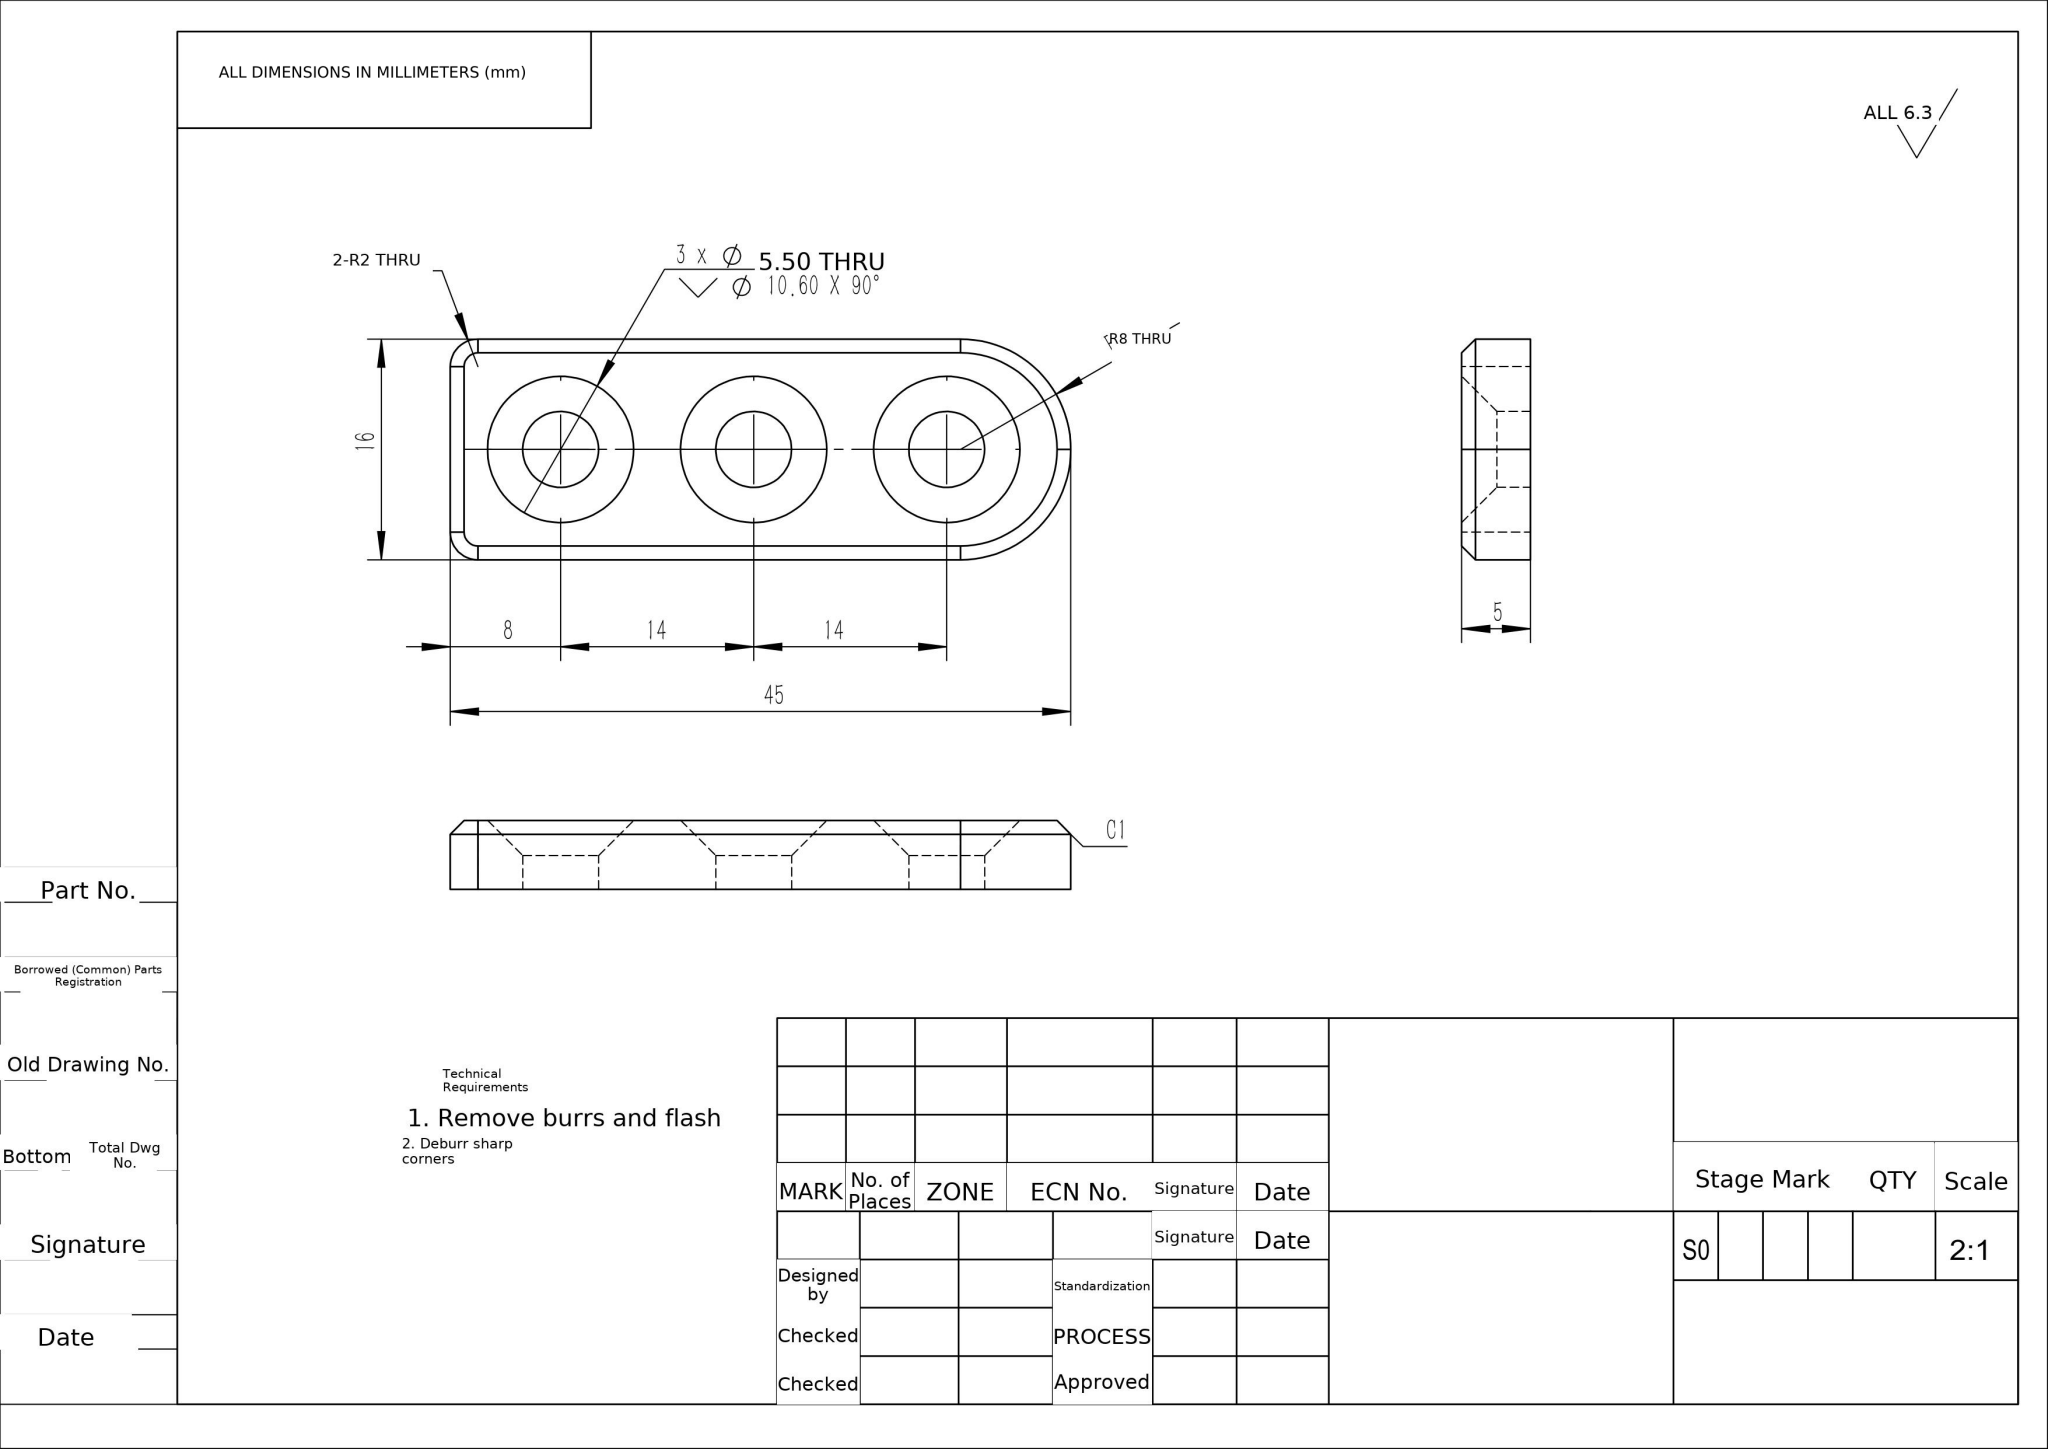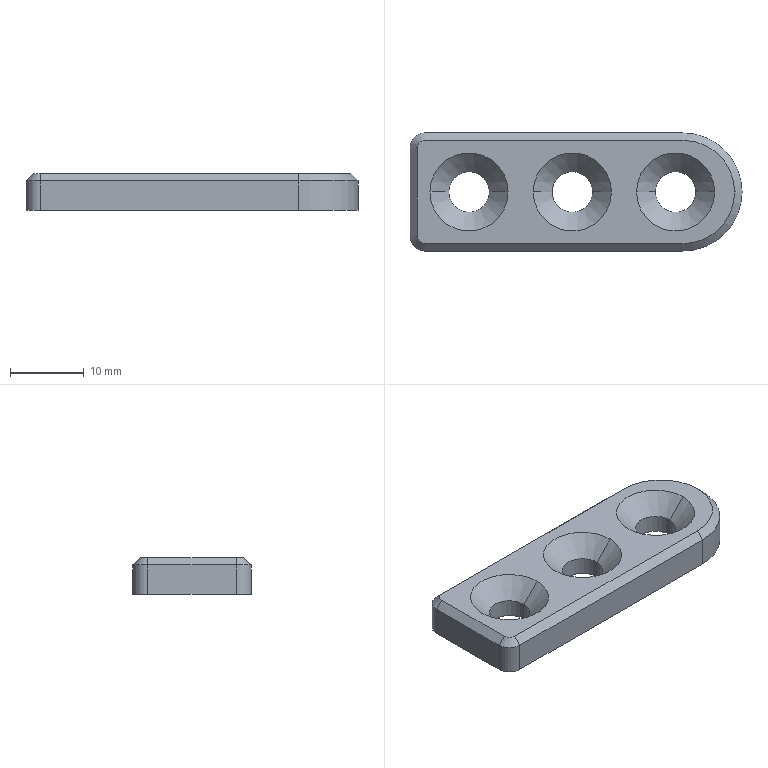Part | NX | mm | 1 solid | 28 faces | box 45 x 16 x 5 mm | volume 2821 mm3 | cone 10 | cylinder 10 | plane 8 | commonest cylinder face diameters 5.5 x6 16 x2 4 x2
STEP:
#1=COLOUR_RGB('',0.502,1.,1.);
#2=FILL_AREA_STYLE_COLOUR('',#1);
#3=FILL_AREA_STYLE('',(#2));
#4=SURFACE_STYLE_FILL_AREA(#3);
#5=SURFACE_SIDE_STYLE('',(#4));
#6=SURFACE_STYLE_USAGE(.BOTH.,#5);
#7=PRESENTATION_STYLE_ASSIGNMENT((#6));
#8=CARTESIAN_POINT('',(5.25,8.,2.45));
#9=VERTEX_POINT('',#8);
#10=CARTESIAN_POINT('',(10.75,8.,2.45));
#11=VERTEX_POINT('',#10);
#12=CARTESIAN_POINT('',(8.,8.,2.45));
#13=DIRECTION('',(0.,0.,1.));
#14=DIRECTION('',(1.,0.,0.));
#15=AXIS2_PLACEMENT_3D('',#12,#13,#14);
#16=CIRCLE('',#15,2.75);
#17=EDGE_CURVE('',#9,#11,#16,.T.);
#18=ORIENTED_EDGE('',*,*,#17,.F.);
#19=CARTESIAN_POINT('',(2.7,8.,5.));
#20=VERTEX_POINT('',#19);
#21=CARTESIAN_POINT('',(2.7,8.,5.));
#22=DIRECTION('',(-0.7071,0.,0.7071));
#23=VECTOR('',#22,1000.);
#24=LINE('',#21,#23);
#25=EDGE_CURVE('',#9,#20,#24,.T.);
#26=ORIENTED_EDGE('',*,*,#25,.T.);
#27=CARTESIAN_POINT('',(13.3,8.,5.));
#28=VERTEX_POINT('',#27);
#29=CARTESIAN_POINT('',(8.,8.,5.));
#30=DIRECTION('',(0.,0.,1.));
#31=DIRECTION('',(1.,0.,0.));
#32=AXIS2_PLACEMENT_3D('',#29,#30,#31);
#33=CIRCLE('',#32,5.3);
#34=EDGE_CURVE('',#20,#28,#33,.T.);
#35=ORIENTED_EDGE('',*,*,#34,.T.);
#36=CARTESIAN_POINT('',(13.3,8.,5.));
#37=DIRECTION('',(0.7071,0.,0.7071));
#38=VECTOR('',#37,1000.);
#39=LINE('',#36,#38);
#40=EDGE_CURVE('',#11,#28,#39,.T.);
#41=ORIENTED_EDGE('',*,*,#40,.F.);
#42=EDGE_LOOP('',(#18,#26,#35,#41));
#43=FACE_OUTER_BOUND('',#42,.T.);
#44=CARTESIAN_POINT('',(8.,8.,5.));
#45=DIRECTION('',(0.,0.,1.));
#46=DIRECTION('',(1.,0.,0.));
#47=AXIS2_PLACEMENT_3D('',#44,#45,#46);
#48=CONICAL_SURFACE('',#47,5.3,0.7854);
#49=ADVANCED_FACE('',(#43),#48,.F.);
#50=CARTESIAN_POINT('',(19.25,8.,2.45));
#51=VERTEX_POINT('',#50);
#52=CARTESIAN_POINT('',(24.75,8.,2.45));
#53=VERTEX_POINT('',#52);
#54=CARTESIAN_POINT('',(22.,8.,2.45));
#55=DIRECTION('',(0.,0.,1.));
#56=DIRECTION('',(1.,0.,0.));
#57=AXIS2_PLACEMENT_3D('',#54,#55,#56);
#58=CIRCLE('',#57,2.75);
#59=EDGE_CURVE('',#51,#53,#58,.T.);
#60=ORIENTED_EDGE('',*,*,#59,.F.);
#61=CARTESIAN_POINT('',(16.7,8.,5.));
#62=VERTEX_POINT('',#61);
#63=CARTESIAN_POINT('',(16.7,8.,5.));
#64=DIRECTION('',(-0.7071,0.,0.7071));
#65=VECTOR('',#64,1000.);
#66=LINE('',#63,#65);
#67=EDGE_CURVE('',#51,#62,#66,.T.);
#68=ORIENTED_EDGE('',*,*,#67,.T.);
#69=CARTESIAN_POINT('',(27.3,8.,5.));
#70=VERTEX_POINT('',#69);
#71=CARTESIAN_POINT('',(22.,8.,5.));
#72=DIRECTION('',(0.,0.,1.));
#73=DIRECTION('',(1.,0.,0.));
#74=AXIS2_PLACEMENT_3D('',#71,#72,#73);
#75=CIRCLE('',#74,5.3);
#76=EDGE_CURVE('',#62,#70,#75,.T.);
#77=ORIENTED_EDGE('',*,*,#76,.T.);
#78=CARTESIAN_POINT('',(27.3,8.,5.));
#79=DIRECTION('',(0.7071,0.,0.7071));
#80=VECTOR('',#79,1000.);
#81=LINE('',#78,#80);
#82=EDGE_CURVE('',#53,#70,#81,.T.);
#83=ORIENTED_EDGE('',*,*,#82,.F.);
#84=EDGE_LOOP('',(#60,#68,#77,#83));
#85=FACE_OUTER_BOUND('',#84,.T.);
#86=CARTESIAN_POINT('',(22.,8.,5.));
#87=DIRECTION('',(0.,0.,1.));
#88=DIRECTION('',(1.,0.,0.));
#89=AXIS2_PLACEMENT_3D('',#86,#87,#88);
#90=CONICAL_SURFACE('',#89,5.3,0.7854);
#91=ADVANCED_FACE('',(#85),#90,.F.);
#92=CARTESIAN_POINT('',(33.25,8.,2.45));
#93=VERTEX_POINT('',#92);
#94=CARTESIAN_POINT('',(38.75,8.,2.45));
#95=VERTEX_POINT('',#94);
#96=CARTESIAN_POINT('',(36.,8.,2.45));
#97=DIRECTION('',(0.,0.,1.));
#98=DIRECTION('',(1.,0.,0.));
#99=AXIS2_PLACEMENT_3D('',#96,#97,#98);
#100=CIRCLE('',#99,2.75);
#101=EDGE_CURVE('',#93,#95,#100,.T.);
#102=ORIENTED_EDGE('',*,*,#101,.F.);
#103=CARTESIAN_POINT('',(30.7,8.,5.));
#104=VERTEX_POINT('',#103);
#105=CARTESIAN_POINT('',(30.7,8.,5.));
#106=DIRECTION('',(-0.7071,0.,0.7071));
#107=VECTOR('',#106,1000.);
#108=LINE('',#105,#107);
#109=EDGE_CURVE('',#93,#104,#108,.T.);
#110=ORIENTED_EDGE('',*,*,#109,.T.);
#111=CARTESIAN_POINT('',(41.3,8.,5.));
#112=VERTEX_POINT('',#111);
#113=CARTESIAN_POINT('',(36.,8.,5.));
#114=DIRECTION('',(0.,0.,1.));
#115=DIRECTION('',(1.,0.,0.));
#116=AXIS2_PLACEMENT_3D('',#113,#114,#115);
#117=CIRCLE('',#116,5.3);
#118=EDGE_CURVE('',#104,#112,#117,.T.);
#119=ORIENTED_EDGE('',*,*,#118,.T.);
#120=CARTESIAN_POINT('',(41.3,8.,5.));
#121=DIRECTION('',(0.7071,0.,0.7071));
#122=VECTOR('',#121,1000.);
#123=LINE('',#120,#122);
#124=EDGE_CURVE('',#95,#112,#123,.T.);
#125=ORIENTED_EDGE('',*,*,#124,.F.);
#126=EDGE_LOOP('',(#102,#110,#119,#125));
#127=FACE_OUTER_BOUND('',#126,.T.);
#128=CARTESIAN_POINT('',(36.,8.,5.));
#129=DIRECTION('',(0.,0.,1.));
#130=DIRECTION('',(1.,0.,0.));
#131=AXIS2_PLACEMENT_3D('',#128,#129,#130);
#132=CONICAL_SURFACE('',#131,5.3,0.7854);
#133=ADVANCED_FACE('',(#127),#132,.F.);
#134=CARTESIAN_POINT('',(33.25,8.,0.));
#135=VERTEX_POINT('',#134);
#136=CARTESIAN_POINT('',(38.75,8.,0.));
#137=VERTEX_POINT('',#136);
#138=CARTESIAN_POINT('',(36.,8.,0.));
#139=DIRECTION('',(0.,0.,1.));
#140=DIRECTION('',(1.,0.,0.));
#141=AXIS2_PLACEMENT_3D('',#138,#139,#140);
#142=CIRCLE('',#141,2.75);
#143=EDGE_CURVE('',#135,#137,#142,.T.);
#144=ORIENTED_EDGE('',*,*,#143,.F.);
#145=CARTESIAN_POINT('',(33.25,8.,0.));
#146=DIRECTION('',(0.,0.,1.));
#147=VECTOR('',#146,1000.);
#148=LINE('',#145,#147);
#149=EDGE_CURVE('',#135,#93,#148,.T.);
#150=ORIENTED_EDGE('',*,*,#149,.T.);
#151=ORIENTED_EDGE('',*,*,#101,.T.);
#152=CARTESIAN_POINT('',(38.75,8.,0.));
#153=DIRECTION('',(0.,0.,1.));
#154=VECTOR('',#153,1000.);
#155=LINE('',#152,#154);
#156=EDGE_CURVE('',#137,#95,#155,.T.);
#157=ORIENTED_EDGE('',*,*,#156,.F.);
#158=EDGE_LOOP('',(#144,#150,#151,#157));
#159=FACE_OUTER_BOUND('',#158,.T.);
#160=CARTESIAN_POINT('',(36.,8.,0.));
#161=DIRECTION('',(0.,0.,1.));
#162=DIRECTION('',(1.,0.,0.));
#163=AXIS2_PLACEMENT_3D('',#160,#161,#162);
#164=CYLINDRICAL_SURFACE('',#163,2.75);
#165=ADVANCED_FACE('',(#159),#164,.F.);
#166=CARTESIAN_POINT('',(19.25,8.,0.));
#167=VERTEX_POINT('',#166);
#168=CARTESIAN_POINT('',(24.75,8.,0.));
#169=VERTEX_POINT('',#168);
#170=CARTESIAN_POINT('',(22.,8.,0.));
#171=DIRECTION('',(0.,0.,1.));
#172=DIRECTION('',(1.,0.,0.));
#173=AXIS2_PLACEMENT_3D('',#170,#171,#172);
#174=CIRCLE('',#173,2.75);
#175=EDGE_CURVE('',#167,#169,#174,.T.);
#176=ORIENTED_EDGE('',*,*,#175,.F.);
#177=CARTESIAN_POINT('',(19.25,8.,0.));
#178=DIRECTION('',(0.,0.,1.));
#179=VECTOR('',#178,1000.);
#180=LINE('',#177,#179);
#181=EDGE_CURVE('',#167,#51,#180,.T.);
#182=ORIENTED_EDGE('',*,*,#181,.T.);
#183=ORIENTED_EDGE('',*,*,#59,.T.);
#184=CARTESIAN_POINT('',(24.75,8.,0.));
#185=DIRECTION('',(0.,0.,1.));
#186=VECTOR('',#185,1000.);
#187=LINE('',#184,#186);
#188=EDGE_CURVE('',#169,#53,#187,.T.);
#189=ORIENTED_EDGE('',*,*,#188,.F.);
#190=EDGE_LOOP('',(#176,#182,#183,#189));
#191=FACE_OUTER_BOUND('',#190,.T.);
#192=CARTESIAN_POINT('',(22.,8.,0.));
#193=DIRECTION('',(0.,0.,1.));
#194=DIRECTION('',(1.,0.,0.));
#195=AXIS2_PLACEMENT_3D('',#192,#193,#194);
#196=CYLINDRICAL_SURFACE('',#195,2.75);
#197=ADVANCED_FACE('',(#191),#196,.F.);
#198=CARTESIAN_POINT('',(5.25,8.,0.));
#199=VERTEX_POINT('',#198);
#200=CARTESIAN_POINT('',(10.75,8.,0.));
#201=VERTEX_POINT('',#200);
#202=CARTESIAN_POINT('',(8.,8.,0.));
#203=DIRECTION('',(0.,0.,1.));
#204=DIRECTION('',(1.,0.,0.));
#205=AXIS2_PLACEMENT_3D('',#202,#203,#204);
#206=CIRCLE('',#205,2.75);
#207=EDGE_CURVE('',#199,#201,#206,.T.);
#208=ORIENTED_EDGE('',*,*,#207,.F.);
#209=CARTESIAN_POINT('',(5.25,8.,0.));
#210=DIRECTION('',(0.,0.,1.));
#211=VECTOR('',#210,1000.);
#212=LINE('',#209,#211);
#213=EDGE_CURVE('',#199,#9,#212,.T.);
#214=ORIENTED_EDGE('',*,*,#213,.T.);
#215=ORIENTED_EDGE('',*,*,#17,.T.);
#216=CARTESIAN_POINT('',(10.75,8.,0.));
#217=DIRECTION('',(0.,0.,1.));
#218=VECTOR('',#217,1000.);
#219=LINE('',#216,#218);
#220=EDGE_CURVE('',#201,#11,#219,.T.);
#221=ORIENTED_EDGE('',*,*,#220,.F.);
#222=EDGE_LOOP('',(#208,#214,#215,#221));
#223=FACE_OUTER_BOUND('',#222,.T.);
#224=CARTESIAN_POINT('',(8.,8.,0.));
#225=DIRECTION('',(0.,0.,1.));
#226=DIRECTION('',(1.,0.,0.));
#227=AXIS2_PLACEMENT_3D('',#224,#225,#226);
#228=CYLINDRICAL_SURFACE('',#227,2.75);
#229=ADVANCED_FACE('',(#223),#228,.F.);
#230=CARTESIAN_POINT('',(0.,2.,0.));
#231=VERTEX_POINT('',#230);
#232=CARTESIAN_POINT('',(0.,2.,4.));
#233=VERTEX_POINT('',#232);
#234=CARTESIAN_POINT('',(0.,2.,5.));
#235=DIRECTION('',(0.,0.,1.));
#236=VECTOR('',#235,1000.);
#237=LINE('',#234,#236);
#238=EDGE_CURVE('',#231,#233,#237,.T.);
#239=ORIENTED_EDGE('',*,*,#238,.T.);
#240=CARTESIAN_POINT('',(0.,14.,4.));
#241=VERTEX_POINT('',#240);
#242=CARTESIAN_POINT('',(0.,0.,4.));
#243=DIRECTION('',(0.,1.,0.));
#244=VECTOR('',#243,1000.);
#245=LINE('',#242,#244);
#246=EDGE_CURVE('',#233,#241,#245,.T.);
#247=ORIENTED_EDGE('',*,*,#246,.T.);
#248=CARTESIAN_POINT('',(0.,14.,0.));
#249=VERTEX_POINT('',#248);
#250=CARTESIAN_POINT('',(0.,14.,5.));
#251=DIRECTION('',(0.,0.,-1.));
#252=VECTOR('',#251,1000.);
#253=LINE('',#250,#252);
#254=EDGE_CURVE('',#241,#249,#253,.T.);
#255=ORIENTED_EDGE('',*,*,#254,.T.);
#256=CARTESIAN_POINT('',(0.,0.,0.));
#257=DIRECTION('',(0.,-1.,0.));
#258=VECTOR('',#257,1000.);
#259=LINE('',#256,#258);
#260=EDGE_CURVE('',#249,#231,#259,.T.);
#261=ORIENTED_EDGE('',*,*,#260,.T.);
#262=EDGE_LOOP('',(#239,#247,#255,#261));
#263=FACE_OUTER_BOUND('',#262,.T.);
#264=CARTESIAN_POINT('',(0.,0.,5.));
#265=DIRECTION('',(1.,0.,0.));
#266=DIRECTION('',(0.,0.,-1.));
#267=AXIS2_PLACEMENT_3D('',#264,#265,#266);
#268=PLANE('',#267);
#269=ADVANCED_FACE('',(#263),#268,.F.);
#270=CARTESIAN_POINT('',(37.,0.,0.));
#271=VERTEX_POINT('',#270);
#272=CARTESIAN_POINT('',(37.,0.,4.));
#273=VERTEX_POINT('',#272);
#274=CARTESIAN_POINT('',(37.,0.,5.));
#275=DIRECTION('',(0.,0.,1.));
#276=VECTOR('',#275,1000.);
#277=LINE('',#274,#276);
#278=EDGE_CURVE('',#271,#273,#277,.T.);
#279=ORIENTED_EDGE('',*,*,#278,.T.);
#280=CARTESIAN_POINT('',(2.,0.,4.));
#281=VERTEX_POINT('',#280);
#282=CARTESIAN_POINT('',(0.,0.,4.));
#283=DIRECTION('',(-1.,0.,0.));
#284=VECTOR('',#283,1000.);
#285=LINE('',#282,#284);
#286=EDGE_CURVE('',#273,#281,#285,.T.);
#287=ORIENTED_EDGE('',*,*,#286,.T.);
#288=CARTESIAN_POINT('',(2.,0.,0.));
#289=VERTEX_POINT('',#288);
#290=CARTESIAN_POINT('',(2.,0.,5.));
#291=DIRECTION('',(0.,0.,-1.));
#292=VECTOR('',#291,1000.);
#293=LINE('',#290,#292);
#294=EDGE_CURVE('',#281,#289,#293,.T.);
#295=ORIENTED_EDGE('',*,*,#294,.T.);
#296=CARTESIAN_POINT('',(0.,0.,0.));
#297=DIRECTION('',(1.,0.,0.));
#298=VECTOR('',#297,1000.);
#299=LINE('',#296,#298);
#300=EDGE_CURVE('',#289,#271,#299,.T.);
#301=ORIENTED_EDGE('',*,*,#300,.T.);
#302=EDGE_LOOP('',(#279,#287,#295,#301));
#303=FACE_OUTER_BOUND('',#302,.T.);
#304=CARTESIAN_POINT('',(0.,0.,5.));
#305=DIRECTION('',(0.,1.,0.));
#306=DIRECTION('',(0.,0.,1.));
#307=AXIS2_PLACEMENT_3D('',#304,#305,#306);
#308=PLANE('',#307);
#309=ADVANCED_FACE('',(#303),#308,.F.);
#310=CARTESIAN_POINT('',(2.,16.,0.));
#311=VERTEX_POINT('',#310);
#312=CARTESIAN_POINT('',(2.,16.,4.));
#313=VERTEX_POINT('',#312);
#314=CARTESIAN_POINT('',(2.,16.,5.));
#315=DIRECTION('',(0.,0.,1.));
#316=VECTOR('',#315,1000.);
#317=LINE('',#314,#316);
#318=EDGE_CURVE('',#311,#313,#317,.T.);
#319=ORIENTED_EDGE('',*,*,#318,.T.);
#320=CARTESIAN_POINT('',(37.,16.,4.));
#321=VERTEX_POINT('',#320);
#322=CARTESIAN_POINT('',(0.,16.,4.));
#323=DIRECTION('',(1.,0.,0.));
#324=VECTOR('',#323,1000.);
#325=LINE('',#322,#324);
#326=EDGE_CURVE('',#313,#321,#325,.T.);
#327=ORIENTED_EDGE('',*,*,#326,.T.);
#328=CARTESIAN_POINT('',(37.,16.,0.));
#329=VERTEX_POINT('',#328);
#330=CARTESIAN_POINT('',(37.,16.,5.));
#331=DIRECTION('',(0.,0.,-1.));
#332=VECTOR('',#331,1000.);
#333=LINE('',#330,#332);
#334=EDGE_CURVE('',#321,#329,#333,.T.);
#335=ORIENTED_EDGE('',*,*,#334,.T.);
#336=CARTESIAN_POINT('',(0.,16.,0.));
#337=DIRECTION('',(-1.,0.,0.));
#338=VECTOR('',#337,1000.);
#339=LINE('',#336,#338);
#340=EDGE_CURVE('',#329,#311,#339,.T.);
#341=ORIENTED_EDGE('',*,*,#340,.T.);
#342=EDGE_LOOP('',(#319,#327,#335,#341));
#343=FACE_OUTER_BOUND('',#342,.T.);
#344=CARTESIAN_POINT('',(0.,16.,5.));
#345=DIRECTION('',(0.,-1.,0.));
#346=DIRECTION('',(0.,0.,-1.));
#347=AXIS2_PLACEMENT_3D('',#344,#345,#346);
#348=PLANE('',#347);
#349=ADVANCED_FACE('',(#343),#348,.F.);
#350=CARTESIAN_POINT('',(8.,8.,5.));
#351=DIRECTION('',(0.,0.,1.));
#352=DIRECTION('',(1.,0.,0.));
#353=AXIS2_PLACEMENT_3D('',#350,#351,#352);
#354=CIRCLE('',#353,5.3);
#355=EDGE_CURVE('',#28,#20,#354,.T.);
#356=ORIENTED_EDGE('',*,*,#355,.F.);
#357=ORIENTED_EDGE('',*,*,#34,.F.);
#358=EDGE_LOOP('',(#356,#357));
#359=FACE_BOUND('',#358,.T.);
#360=CARTESIAN_POINT('',(22.,8.,5.));
#361=DIRECTION('',(0.,0.,1.));
#362=DIRECTION('',(1.,0.,0.));
#363=AXIS2_PLACEMENT_3D('',#360,#361,#362);
#364=CIRCLE('',#363,5.3);
#365=EDGE_CURVE('',#70,#62,#364,.T.);
#366=ORIENTED_EDGE('',*,*,#365,.F.);
#367=ORIENTED_EDGE('',*,*,#76,.F.);
#368=EDGE_LOOP('',(#366,#367));
#369=FACE_BOUND('',#368,.T.);
#370=CARTESIAN_POINT('',(36.,8.,5.));
#371=DIRECTION('',(0.,0.,1.));
#372=DIRECTION('',(1.,0.,0.));
#373=AXIS2_PLACEMENT_3D('',#370,#371,#372);
#374=CIRCLE('',#373,5.3);
#375=EDGE_CURVE('',#112,#104,#374,.T.);
#376=ORIENTED_EDGE('',*,*,#375,.F.);
#377=ORIENTED_EDGE('',*,*,#118,.F.);
#378=EDGE_LOOP('',(#376,#377));
#379=FACE_BOUND('',#378,.T.);
#380=CARTESIAN_POINT('',(2.,15.,5.));
#381=VERTEX_POINT('',#380);
#382=CARTESIAN_POINT('',(1.,14.,5.));
#383=VERTEX_POINT('',#382);
#384=CARTESIAN_POINT('',(2.,14.,5.));
#385=DIRECTION('',(0.,0.,1.));
#386=DIRECTION('',(-1.,0.,0.));
#387=AXIS2_PLACEMENT_3D('',#384,#385,#386);
#388=CIRCLE('',#387,1.);
#389=EDGE_CURVE('',#381,#383,#388,.T.);
#390=ORIENTED_EDGE('',*,*,#389,.T.);
#391=CARTESIAN_POINT('',(1.,2.,5.));
#392=VERTEX_POINT('',#391);
#393=CARTESIAN_POINT('',(1.,0.,5.));
#394=DIRECTION('',(0.,-1.,0.));
#395=VECTOR('',#394,1000.);
#396=LINE('',#393,#395);
#397=EDGE_CURVE('',#383,#392,#396,.T.);
#398=ORIENTED_EDGE('',*,*,#397,.T.);
#399=CARTESIAN_POINT('',(2.,1.,5.));
#400=VERTEX_POINT('',#399);
#401=CARTESIAN_POINT('',(2.,2.,5.));
#402=DIRECTION('',(0.,0.,1.));
#403=DIRECTION('',(-1.,0.,0.));
#404=AXIS2_PLACEMENT_3D('',#401,#402,#403);
#405=CIRCLE('',#404,1.);
#406=EDGE_CURVE('',#392,#400,#405,.T.);
#407=ORIENTED_EDGE('',*,*,#406,.T.);
#408=CARTESIAN_POINT('',(37.,1.,5.));
#409=VERTEX_POINT('',#408);
#410=CARTESIAN_POINT('',(0.,1.,5.));
#411=DIRECTION('',(1.,0.,0.));
#412=VECTOR('',#411,1000.);
#413=LINE('',#410,#412);
#414=EDGE_CURVE('',#400,#409,#413,.T.);
#415=ORIENTED_EDGE('',*,*,#414,.T.);
#416=CARTESIAN_POINT('',(44.,8.,5.));
#417=VERTEX_POINT('',#416);
#418=CARTESIAN_POINT('',(37.,8.,5.));
#419=DIRECTION('',(0.,0.,1.));
#420=DIRECTION('',(-1.,0.,0.));
#421=AXIS2_PLACEMENT_3D('',#418,#419,#420);
#422=CIRCLE('',#421,7.);
#423=EDGE_CURVE('',#409,#417,#422,.T.);
#424=ORIENTED_EDGE('',*,*,#423,.T.);
#425=CARTESIAN_POINT('',(37.,15.,5.));
#426=VERTEX_POINT('',#425);
#427=CARTESIAN_POINT('',(37.,8.,5.));
#428=DIRECTION('',(0.,0.,1.));
#429=DIRECTION('',(-1.,0.,0.));
#430=AXIS2_PLACEMENT_3D('',#427,#428,#429);
#431=CIRCLE('',#430,7.);
#432=EDGE_CURVE('',#417,#426,#431,.T.);
#433=ORIENTED_EDGE('',*,*,#432,.T.);
#434=CARTESIAN_POINT('',(0.,15.,5.));
#435=DIRECTION('',(-1.,0.,0.));
#436=VECTOR('',#435,1000.);
#437=LINE('',#434,#436);
#438=EDGE_CURVE('',#426,#381,#437,.T.);
#439=ORIENTED_EDGE('',*,*,#438,.T.);
#440=EDGE_LOOP('',(#390,#398,#407,#415,#424,#433,#439));
#441=FACE_OUTER_BOUND('',#440,.T.);
#442=CARTESIAN_POINT('',(0.,0.,5.));
#443=DIRECTION('',(0.,0.,-1.));
#444=DIRECTION('',(-1.,0.,0.));
#445=AXIS2_PLACEMENT_3D('',#442,#443,#444);
#446=PLANE('',#445);
#447=ADVANCED_FACE('',(#359,#369,#379,#441),#446,.F.);
#448=CARTESIAN_POINT('',(36.,8.,0.));
#449=DIRECTION('',(0.,0.,1.));
#450=DIRECTION('',(1.,0.,0.));
#451=AXIS2_PLACEMENT_3D('',#448,#449,#450);
#452=CIRCLE('',#451,2.75);
#453=EDGE_CURVE('',#137,#135,#452,.T.);
#454=ORIENTED_EDGE('',*,*,#453,.T.);
#455=ORIENTED_EDGE('',*,*,#143,.T.);
#456=EDGE_LOOP('',(#454,#455));
#457=FACE_BOUND('',#456,.T.);
#458=CARTESIAN_POINT('',(22.,8.,0.));
#459=DIRECTION('',(0.,0.,1.));
#460=DIRECTION('',(1.,0.,0.));
#461=AXIS2_PLACEMENT_3D('',#458,#459,#460);
#462=CIRCLE('',#461,2.75);
#463=EDGE_CURVE('',#169,#167,#462,.T.);
#464=ORIENTED_EDGE('',*,*,#463,.T.);
#465=ORIENTED_EDGE('',*,*,#175,.T.);
#466=EDGE_LOOP('',(#464,#465));
#467=FACE_BOUND('',#466,.T.);
#468=CARTESIAN_POINT('',(8.,8.,0.));
#469=DIRECTION('',(0.,0.,1.));
#470=DIRECTION('',(1.,0.,0.));
#471=AXIS2_PLACEMENT_3D('',#468,#469,#470);
#472=CIRCLE('',#471,2.75);
#473=EDGE_CURVE('',#201,#199,#472,.T.);
#474=ORIENTED_EDGE('',*,*,#473,.T.);
#475=ORIENTED_EDGE('',*,*,#207,.T.);
#476=EDGE_LOOP('',(#474,#475));
#477=FACE_BOUND('',#476,.T.);
#478=ORIENTED_EDGE('',*,*,#300,.F.);
#479=CARTESIAN_POINT('',(2.,2.,0.));
#480=DIRECTION('',(0.,0.,-1.));
#481=DIRECTION('',(-1.,0.,0.));
#482=AXIS2_PLACEMENT_3D('',#479,#480,#481);
#483=CIRCLE('',#482,2.);
#484=EDGE_CURVE('',#289,#231,#483,.T.);
#485=ORIENTED_EDGE('',*,*,#484,.T.);
#486=ORIENTED_EDGE('',*,*,#260,.F.);
#487=CARTESIAN_POINT('',(2.,14.,0.));
#488=DIRECTION('',(0.,0.,-1.));
#489=DIRECTION('',(-1.,0.,0.));
#490=AXIS2_PLACEMENT_3D('',#487,#488,#489);
#491=CIRCLE('',#490,2.);
#492=EDGE_CURVE('',#249,#311,#491,.T.);
#493=ORIENTED_EDGE('',*,*,#492,.T.);
#494=ORIENTED_EDGE('',*,*,#340,.F.);
#495=CARTESIAN_POINT('',(45.,8.,0.));
#496=VERTEX_POINT('',#495);
#497=CARTESIAN_POINT('',(37.,8.,0.));
#498=DIRECTION('',(0.,0.,-1.));
#499=DIRECTION('',(-1.,0.,0.));
#500=AXIS2_PLACEMENT_3D('',#497,#498,#499);
#501=CIRCLE('',#500,8.);
#502=EDGE_CURVE('',#329,#496,#501,.T.);
#503=ORIENTED_EDGE('',*,*,#502,.T.);
#504=CARTESIAN_POINT('',(37.,8.,0.));
#505=DIRECTION('',(0.,0.,-1.));
#506=DIRECTION('',(-1.,0.,0.));
#507=AXIS2_PLACEMENT_3D('',#504,#505,#506);
#508=CIRCLE('',#507,8.);
#509=EDGE_CURVE('',#496,#271,#508,.T.);
#510=ORIENTED_EDGE('',*,*,#509,.T.);
#511=EDGE_LOOP('',(#478,#485,#486,#493,#494,#503,#510));
#512=FACE_OUTER_BOUND('',#511,.T.);
#513=CARTESIAN_POINT('',(0.,0.,0.));
#514=DIRECTION('',(0.,0.,-1.));
#515=DIRECTION('',(-1.,0.,0.));
#516=AXIS2_PLACEMENT_3D('',#513,#514,#515);
#517=PLANE('',#516);
#518=ADVANCED_FACE('',(#457,#467,#477,#512),#517,.T.);
#519=ORIENTED_EDGE('',*,*,#334,.F.);
#520=CARTESIAN_POINT('',(45.,8.,4.));
#521=VERTEX_POINT('',#520);
#522=CARTESIAN_POINT('',(37.,8.,4.));
#523=DIRECTION('',(0.,0.,-1.));
#524=DIRECTION('',(-1.,0.,0.));
#525=AXIS2_PLACEMENT_3D('',#522,#523,#524);
#526=CIRCLE('',#525,8.);
#527=EDGE_CURVE('',#321,#521,#526,.T.);
#528=ORIENTED_EDGE('',*,*,#527,.T.);
#529=CARTESIAN_POINT('',(45.,8.,5.));
#530=DIRECTION('',(0.,0.,1.));
#531=VECTOR('',#530,1000.);
#532=LINE('',#529,#531);
#533=EDGE_CURVE('',#496,#521,#532,.T.);
#534=ORIENTED_EDGE('',*,*,#533,.F.);
#535=ORIENTED_EDGE('',*,*,#502,.F.);
#536=EDGE_LOOP('',(#519,#528,#534,#535));
#537=FACE_OUTER_BOUND('',#536,.T.);
#538=CARTESIAN_POINT('',(37.,8.,5.));
#539=DIRECTION('',(0.,0.,-1.));
#540=DIRECTION('',(-1.,0.,0.));
#541=AXIS2_PLACEMENT_3D('',#538,#539,#540);
#542=CYLINDRICAL_SURFACE('',#541,8.);
#543=ADVANCED_FACE('',(#537),#542,.T.);
#544=ORIENTED_EDGE('',*,*,#533,.T.);
#545=CARTESIAN_POINT('',(37.,8.,4.));
#546=DIRECTION('',(0.,0.,-1.));
#547=DIRECTION('',(-1.,0.,0.));
#548=AXIS2_PLACEMENT_3D('',#545,#546,#547);
#549=CIRCLE('',#548,8.);
#550=EDGE_CURVE('',#521,#273,#549,.T.);
#551=ORIENTED_EDGE('',*,*,#550,.T.);
#552=ORIENTED_EDGE('',*,*,#278,.F.);
#553=ORIENTED_EDGE('',*,*,#509,.F.);
#554=EDGE_LOOP('',(#544,#551,#552,#553));
#555=FACE_OUTER_BOUND('',#554,.T.);
#556=CARTESIAN_POINT('',(37.,8.,5.));
#557=DIRECTION('',(0.,0.,-1.));
#558=DIRECTION('',(-1.,0.,0.));
#559=AXIS2_PLACEMENT_3D('',#556,#557,#558);
#560=CYLINDRICAL_SURFACE('',#559,8.);
#561=ADVANCED_FACE('',(#555),#560,.T.);
#562=ORIENTED_EDGE('',*,*,#294,.F.);
#563=CARTESIAN_POINT('',(2.,2.,4.));
#564=DIRECTION('',(0.,0.,-1.));
#565=DIRECTION('',(-1.,0.,0.));
#566=AXIS2_PLACEMENT_3D('',#563,#564,#565);
#567=CIRCLE('',#566,2.);
#568=EDGE_CURVE('',#281,#233,#567,.T.);
#569=ORIENTED_EDGE('',*,*,#568,.T.);
#570=ORIENTED_EDGE('',*,*,#238,.F.);
#571=ORIENTED_EDGE('',*,*,#484,.F.);
#572=EDGE_LOOP('',(#562,#569,#570,#571));
#573=FACE_OUTER_BOUND('',#572,.T.);
#574=CARTESIAN_POINT('',(2.,2.,5.));
#575=DIRECTION('',(0.,0.,-1.));
#576=DIRECTION('',(-1.,0.,0.));
#577=AXIS2_PLACEMENT_3D('',#574,#575,#576);
#578=CYLINDRICAL_SURFACE('',#577,2.);
#579=ADVANCED_FACE('',(#573),#578,.T.);
#580=ORIENTED_EDGE('',*,*,#254,.F.);
#581=CARTESIAN_POINT('',(2.,14.,4.));
#582=DIRECTION('',(0.,0.,-1.));
#583=DIRECTION('',(-1.,0.,0.));
#584=AXIS2_PLACEMENT_3D('',#581,#582,#583);
#585=CIRCLE('',#584,2.);
#586=EDGE_CURVE('',#241,#313,#585,.T.);
#587=ORIENTED_EDGE('',*,*,#586,.T.);
#588=ORIENTED_EDGE('',*,*,#318,.F.);
#589=ORIENTED_EDGE('',*,*,#492,.F.);
#590=EDGE_LOOP('',(#580,#587,#588,#589));
#591=FACE_OUTER_BOUND('',#590,.T.);
#592=CARTESIAN_POINT('',(2.,14.,5.));
#593=DIRECTION('',(0.,0.,-1.));
#594=DIRECTION('',(-1.,0.,0.));
#595=AXIS2_PLACEMENT_3D('',#592,#593,#594);
#596=CYLINDRICAL_SURFACE('',#595,2.);
#597=ADVANCED_FACE('',(#591),#596,.T.);
#598=ORIENTED_EDGE('',*,*,#213,.F.);
#599=ORIENTED_EDGE('',*,*,#473,.F.);
#600=ORIENTED_EDGE('',*,*,#220,.T.);
#601=CARTESIAN_POINT('',(8.,8.,2.45));
#602=DIRECTION('',(0.,0.,1.));
#603=DIRECTION('',(1.,0.,0.));
#604=AXIS2_PLACEMENT_3D('',#601,#602,#603);
#605=CIRCLE('',#604,2.75);
#606=EDGE_CURVE('',#11,#9,#605,.T.);
#607=ORIENTED_EDGE('',*,*,#606,.T.);
#608=EDGE_LOOP('',(#598,#599,#600,#607));
#609=FACE_OUTER_BOUND('',#608,.T.);
#610=CARTESIAN_POINT('',(8.,8.,0.));
#611=DIRECTION('',(0.,0.,1.));
#612=DIRECTION('',(1.,0.,0.));
#613=AXIS2_PLACEMENT_3D('',#610,#611,#612);
#614=CYLINDRICAL_SURFACE('',#613,2.75);
#615=ADVANCED_FACE('',(#609),#614,.F.);
#616=ORIENTED_EDGE('',*,*,#181,.F.);
#617=ORIENTED_EDGE('',*,*,#463,.F.);
#618=ORIENTED_EDGE('',*,*,#188,.T.);
#619=CARTESIAN_POINT('',(22.,8.,2.45));
#620=DIRECTION('',(0.,0.,1.));
#621=DIRECTION('',(1.,0.,0.));
#622=AXIS2_PLACEMENT_3D('',#619,#620,#621);
#623=CIRCLE('',#622,2.75);
#624=EDGE_CURVE('',#53,#51,#623,.T.);
#625=ORIENTED_EDGE('',*,*,#624,.T.);
#626=EDGE_LOOP('',(#616,#617,#618,#625));
#627=FACE_OUTER_BOUND('',#626,.T.);
#628=CARTESIAN_POINT('',(22.,8.,0.));
#629=DIRECTION('',(0.,0.,1.));
#630=DIRECTION('',(1.,0.,0.));
#631=AXIS2_PLACEMENT_3D('',#628,#629,#630);
#632=CYLINDRICAL_SURFACE('',#631,2.75);
#633=ADVANCED_FACE('',(#627),#632,.F.);
#634=ORIENTED_EDGE('',*,*,#149,.F.);
#635=ORIENTED_EDGE('',*,*,#453,.F.);
#636=ORIENTED_EDGE('',*,*,#156,.T.);
#637=CARTESIAN_POINT('',(36.,8.,2.45));
#638=DIRECTION('',(0.,0.,1.));
#639=DIRECTION('',(1.,0.,0.));
#640=AXIS2_PLACEMENT_3D('',#637,#638,#639);
#641=CIRCLE('',#640,2.75);
#642=EDGE_CURVE('',#95,#93,#641,.T.);
#643=ORIENTED_EDGE('',*,*,#642,.T.);
#644=EDGE_LOOP('',(#634,#635,#636,#643));
#645=FACE_OUTER_BOUND('',#644,.T.);
#646=CARTESIAN_POINT('',(36.,8.,0.));
#647=DIRECTION('',(0.,0.,1.));
#648=DIRECTION('',(1.,0.,0.));
#649=AXIS2_PLACEMENT_3D('',#646,#647,#648);
#650=CYLINDRICAL_SURFACE('',#649,2.75);
#651=ADVANCED_FACE('',(#645),#650,.F.);
#652=CARTESIAN_POINT('',(37.,15.,5.));
#653=DIRECTION('',(0.,0.7071,-0.7071));
#654=VECTOR('',#653,1000.);
#655=LINE('',#652,#654);
#656=EDGE_CURVE('',#426,#321,#655,.T.);
#657=ORIENTED_EDGE('',*,*,#656,.F.);
#658=ORIENTED_EDGE('',*,*,#432,.F.);
#659=CARTESIAN_POINT('',(45.,8.,4.));
#660=DIRECTION('',(-0.7071,0.,0.7071));
#661=VECTOR('',#660,1000.);
#662=LINE('',#659,#661);
#663=EDGE_CURVE('',#521,#417,#662,.T.);
#664=ORIENTED_EDGE('',*,*,#663,.F.);
#665=ORIENTED_EDGE('',*,*,#527,.F.);
#666=EDGE_LOOP('',(#657,#658,#664,#665));
#667=FACE_OUTER_BOUND('',#666,.T.);
#668=CARTESIAN_POINT('',(37.,8.,5.));
#669=DIRECTION('',(0.,0.,-1.));
#670=DIRECTION('',(-1.,0.,0.));
#671=AXIS2_PLACEMENT_3D('',#668,#669,#670);
#672=CONICAL_SURFACE('',#671,7.,0.7854);
#673=ADVANCED_FACE('',(#667),#672,.T.);
#674=ORIENTED_EDGE('',*,*,#663,.T.);
#675=ORIENTED_EDGE('',*,*,#423,.F.);
#676=CARTESIAN_POINT('',(37.,0.,4.));
#677=DIRECTION('',(0.,0.7071,0.7071));
#678=VECTOR('',#677,1000.);
#679=LINE('',#676,#678);
#680=EDGE_CURVE('',#273,#409,#679,.T.);
#681=ORIENTED_EDGE('',*,*,#680,.F.);
#682=ORIENTED_EDGE('',*,*,#550,.F.);
#683=EDGE_LOOP('',(#674,#675,#681,#682));
#684=FACE_OUTER_BOUND('',#683,.T.);
#685=CARTESIAN_POINT('',(37.,8.,5.));
#686=DIRECTION('',(0.,0.,-1.));
#687=DIRECTION('',(-1.,0.,0.));
#688=AXIS2_PLACEMENT_3D('',#685,#686,#687);
#689=CONICAL_SURFACE('',#688,7.,0.7854);
#690=ADVANCED_FACE('',(#684),#689,.T.);
#691=ORIENTED_EDGE('',*,*,#656,.T.);
#692=ORIENTED_EDGE('',*,*,#326,.F.);
#693=CARTESIAN_POINT('',(2.,15.,5.));
#694=DIRECTION('',(0.,0.7071,-0.7071));
#695=VECTOR('',#694,1000.);
#696=LINE('',#693,#695);
#697=EDGE_CURVE('',#381,#313,#696,.T.);
#698=ORIENTED_EDGE('',*,*,#697,.F.);
#699=ORIENTED_EDGE('',*,*,#438,.F.);
#700=EDGE_LOOP('',(#691,#692,#698,#699));
#701=FACE_OUTER_BOUND('',#700,.T.);
#702=CARTESIAN_POINT('',(0.,15.,5.));
#703=DIRECTION('',(0.,-0.7071,-0.7071));
#704=DIRECTION('',(-1.,0.,0.));
#705=AXIS2_PLACEMENT_3D('',#702,#703,#704);
#706=PLANE('',#705);
#707=ADVANCED_FACE('',(#701),#706,.F.);
#708=ORIENTED_EDGE('',*,*,#680,.T.);
#709=ORIENTED_EDGE('',*,*,#414,.F.);
#710=CARTESIAN_POINT('',(2.,0.,4.));
#711=DIRECTION('',(0.,0.7071,0.7071));
#712=VECTOR('',#711,1000.);
#713=LINE('',#710,#712);
#714=EDGE_CURVE('',#281,#400,#713,.T.);
#715=ORIENTED_EDGE('',*,*,#714,.F.);
#716=ORIENTED_EDGE('',*,*,#286,.F.);
#717=EDGE_LOOP('',(#708,#709,#715,#716));
#718=FACE_OUTER_BOUND('',#717,.T.);
#719=CARTESIAN_POINT('',(0.,1.,5.));
#720=DIRECTION('',(0.,0.7071,-0.7071));
#721=DIRECTION('',(1.,0.,0.));
#722=AXIS2_PLACEMENT_3D('',#719,#720,#721);
#723=PLANE('',#722);
#724=ADVANCED_FACE('',(#718),#723,.F.);
#725=ORIENTED_EDGE('',*,*,#697,.T.);
#726=ORIENTED_EDGE('',*,*,#586,.F.);
#727=CARTESIAN_POINT('',(1.,14.,5.));
#728=DIRECTION('',(-0.7071,0.,-0.7071));
#729=VECTOR('',#728,1000.);
#730=LINE('',#727,#729);
#731=EDGE_CURVE('',#383,#241,#730,.T.);
#732=ORIENTED_EDGE('',*,*,#731,.F.);
#733=ORIENTED_EDGE('',*,*,#389,.F.);
#734=EDGE_LOOP('',(#725,#726,#732,#733));
#735=FACE_OUTER_BOUND('',#734,.T.);
#736=CARTESIAN_POINT('',(2.,14.,5.));
#737=DIRECTION('',(0.,0.,-1.));
#738=DIRECTION('',(-1.,0.,0.));
#739=AXIS2_PLACEMENT_3D('',#736,#737,#738);
#740=CONICAL_SURFACE('',#739,1.,0.7854);
#741=ADVANCED_FACE('',(#735),#740,.T.);
#742=ORIENTED_EDGE('',*,*,#714,.T.);
#743=ORIENTED_EDGE('',*,*,#406,.F.);
#744=CARTESIAN_POINT('',(0.,2.,4.));
#745=DIRECTION('',(0.7071,0.,0.7071));
#746=VECTOR('',#745,1000.);
#747=LINE('',#744,#746);
#748=EDGE_CURVE('',#233,#392,#747,.T.);
#749=ORIENTED_EDGE('',*,*,#748,.F.);
#750=ORIENTED_EDGE('',*,*,#568,.F.);
#751=EDGE_LOOP('',(#742,#743,#749,#750));
#752=FACE_OUTER_BOUND('',#751,.T.);
#753=CARTESIAN_POINT('',(2.,2.,5.));
#754=DIRECTION('',(0.,0.,-1.));
#755=DIRECTION('',(-1.,0.,0.));
#756=AXIS2_PLACEMENT_3D('',#753,#754,#755);
#757=CONICAL_SURFACE('',#756,1.,0.7854);
#758=ADVANCED_FACE('',(#752),#757,.T.);
#759=ORIENTED_EDGE('',*,*,#731,.T.);
#760=ORIENTED_EDGE('',*,*,#246,.F.);
#761=ORIENTED_EDGE('',*,*,#748,.T.);
#762=ORIENTED_EDGE('',*,*,#397,.F.);
#763=EDGE_LOOP('',(#759,#760,#761,#762));
#764=FACE_OUTER_BOUND('',#763,.T.);
#765=CARTESIAN_POINT('',(1.,0.,5.));
#766=DIRECTION('',(0.7071,0.,-0.7071));
#767=DIRECTION('',(0.,-1.,0.));
#768=AXIS2_PLACEMENT_3D('',#765,#766,#767);
#769=PLANE('',#768);
#770=ADVANCED_FACE('',(#764),#769,.F.);
#771=ORIENTED_EDGE('',*,*,#109,.F.);
#772=ORIENTED_EDGE('',*,*,#642,.F.);
#773=ORIENTED_EDGE('',*,*,#124,.T.);
#774=ORIENTED_EDGE('',*,*,#375,.T.);
#775=EDGE_LOOP('',(#771,#772,#773,#774));
#776=FACE_OUTER_BOUND('',#775,.T.);
#777=CARTESIAN_POINT('',(36.,8.,5.));
#778=DIRECTION('',(0.,0.,1.));
#779=DIRECTION('',(1.,0.,0.));
#780=AXIS2_PLACEMENT_3D('',#777,#778,#779);
#781=CONICAL_SURFACE('',#780,5.3,0.7854);
#782=ADVANCED_FACE('',(#776),#781,.F.);
#783=ORIENTED_EDGE('',*,*,#67,.F.);
#784=ORIENTED_EDGE('',*,*,#624,.F.);
#785=ORIENTED_EDGE('',*,*,#82,.T.);
#786=ORIENTED_EDGE('',*,*,#365,.T.);
#787=EDGE_LOOP('',(#783,#784,#785,#786));
#788=FACE_OUTER_BOUND('',#787,.T.);
#789=CARTESIAN_POINT('',(22.,8.,5.));
#790=DIRECTION('',(0.,0.,1.));
#791=DIRECTION('',(1.,0.,0.));
#792=AXIS2_PLACEMENT_3D('',#789,#790,#791);
#793=CONICAL_SURFACE('',#792,5.3,0.7854);
#794=ADVANCED_FACE('',(#788),#793,.F.);
#795=ORIENTED_EDGE('',*,*,#25,.F.);
#796=ORIENTED_EDGE('',*,*,#606,.F.);
#797=ORIENTED_EDGE('',*,*,#40,.T.);
#798=ORIENTED_EDGE('',*,*,#355,.T.);
#799=EDGE_LOOP('',(#795,#796,#797,#798));
#800=FACE_OUTER_BOUND('',#799,.T.);
#801=CARTESIAN_POINT('',(8.,8.,5.));
#802=DIRECTION('',(0.,0.,1.));
#803=DIRECTION('',(1.,0.,0.));
#804=AXIS2_PLACEMENT_3D('',#801,#802,#803);
#805=CONICAL_SURFACE('',#804,5.3,0.7854);
#806=ADVANCED_FACE('',(#800),#805,.F.);
#807=CLOSED_SHELL('',(#49,#91,#133,#165,#197,#229,#269,#309,#349,#447,#518,#543,#561,#579,#597,#615,#633,#651,#673,#690,#707,#724,#741,#758,#770,#782,#794,#806));
#808=MANIFOLD_SOLID_BREP('',#807);
#809=CARTESIAN_POINT('',(0.,0.,0.));
#810=DIRECTION('',(0.,0.,1.));
#811=DIRECTION('',(1.,0.,0.));
#812=AXIS2_PLACEMENT_3D('',#809,#810,#811);
#813=(LENGTH_UNIT()NAMED_UNIT(*)SI_UNIT(.MILLI.,.METRE.));
#814=UNCERTAINTY_MEASURE_WITH_UNIT(LENGTH_MEASURE(0.00001),#813,'','');
#815=(NAMED_UNIT(*)PLANE_ANGLE_UNIT()SI_UNIT($,.RADIAN.));
#816=(NAMED_UNIT(*)SI_UNIT($,.STERADIAN.)SOLID_ANGLE_UNIT());
#817=(GEOMETRIC_REPRESENTATION_CONTEXT(3)GLOBAL_UNCERTAINTY_ASSIGNED_CONTEXT((#814))GLOBAL_UNIT_ASSIGNED_CONTEXT((#813,#815,#816))REPRESENTATION_CONTEXT('',''));
#818=ADVANCED_BREP_SHAPE_REPRESENTATION('',(#808,#812),#817);
#819=STYLED_ITEM('',(#7),#818);
#820=(LENGTH_UNIT()NAMED_UNIT(*)SI_UNIT(.MILLI.,.METRE.));
#821=UNCERTAINTY_MEASURE_WITH_UNIT(LENGTH_MEASURE(0.00001),#820,'','');
#822=(NAMED_UNIT(*)PLANE_ANGLE_UNIT()SI_UNIT($,.RADIAN.));
#823=(NAMED_UNIT(*)SI_UNIT($,.STERADIAN.)SOLID_ANGLE_UNIT());
#824=(GEOMETRIC_REPRESENTATION_CONTEXT(3)GLOBAL_UNCERTAINTY_ASSIGNED_CONTEXT((#821))GLOBAL_UNIT_ASSIGNED_CONTEXT((#820,#822,#823))REPRESENTATION_CONTEXT('',''));
#825=MECHANICAL_DESIGN_GEOMETRIC_PRESENTATION_REPRESENTATION('',(#819),#824);
#826=PRESENTATION_LAYER_ASSIGNMENT('','',(#819));
#827=COLOUR_RGB('',0.502,1.,1.);
#828=FILL_AREA_STYLE_COLOUR('',#827);
#829=FILL_AREA_STYLE('',(#828));
#830=SURFACE_STYLE_FILL_AREA(#829);
#831=SURFACE_SIDE_STYLE('',(#830));
#832=SURFACE_STYLE_USAGE(.BOTH.,#831);
#833=PRESENTATION_STYLE_ASSIGNMENT((#832));
#834=STYLED_ITEM('',(#833),#808);
#835=(LENGTH_UNIT()NAMED_UNIT(*)SI_UNIT(.MILLI.,.METRE.));
#836=UNCERTAINTY_MEASURE_WITH_UNIT(LENGTH_MEASURE(0.00001),#835,'','');
#837=(NAMED_UNIT(*)PLANE_ANGLE_UNIT()SI_UNIT($,.RADIAN.));
#838=(NAMED_UNIT(*)SI_UNIT($,.STERADIAN.)SOLID_ANGLE_UNIT());
#839=(GEOMETRIC_REPRESENTATION_CONTEXT(3)GLOBAL_UNCERTAINTY_ASSIGNED_CONTEXT((#836))GLOBAL_UNIT_ASSIGNED_CONTEXT((#835,#837,#838))REPRESENTATION_CONTEXT('',''));
#840=MECHANICAL_DESIGN_GEOMETRIC_PRESENTATION_REPRESENTATION('',(#834),#839);
#841=PRESENTATION_LAYER_ASSIGNMENT('','',(#834));